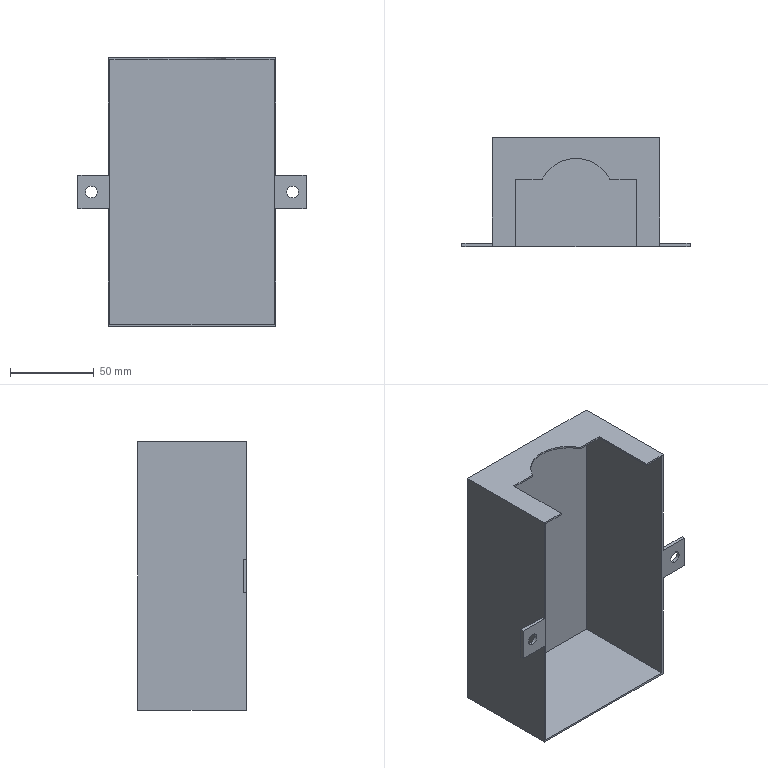Component | SolidWorks | OT-0100-029(CylinderGuard)-1 | 1 solid | 28 faces | box 136 x 65 x 160 mm | volume 47070 mm3 | plane 23 | cylinder 5 | commonest cylinder face diameters 7 x4 45 x1
build123d program:
from build123d import *

# Parameters (mm, degrees)
SKETCH1_W           = 100
SKETCH1_H           = 160
BOSS_EXTRUDE1_DEPTH = 65
SHELL1_T            = -1
SKETCH2_W           = 18
SKETCH2_H           = 20
SKETCH2_R           = 3.5
BOSS_EXTRUDE2_DEPTH = 2
CUT_EXTRUDE1_REACH  = 187.604
CUT_EXTRUDE2_START  = -1
SKETCH4_W           = 72
SKETCH4_H           = 40
CUT_EXTRUDE2_DEPTH  = 1


with BuildPart() as part:
    # Sketch1 → Boss-Extrude1 (new body)
    with BuildSketch(Plane(origin=(0, 0, 0), x_dir=(1, 0, 0), z_dir=(0, 1, 0))):
        Rectangle(SKETCH1_W, SKETCH1_H)
    extrude(amount=-BOSS_EXTRUDE1_DEPTH)

    # Shell1
    shell1_openings = [part.faces().sort_by_distance(p)[0] for p in [
        (0, -65, 0),
    ]]
    offset(amount=SHELL1_T, openings=shell1_openings, kind=Kind.INTERSECTION)

    # Sketch2 → Boss-Extrude2 (add)
    # profile 1 of 2: a face of its own
    with BuildSketch(Plane.XZ.offset(65)):
        with Locations((59, 0)):
            Rectangle(SKETCH2_W, SKETCH2_H)
        with Locations(Location((60, 0, 0), (0, 0, 270))):
            Circle(SKETCH2_R, mode=Mode.SUBTRACT)
    # profile 2 of 2: a face of its own
    with BuildSketch(Plane.XZ.offset(65)):
        with Locations((-59, 0)):
            Rectangle(SKETCH2_W, SKETCH2_H)
        with Locations(Location((-60, 0, 0), (0, 0, 90))):
            Circle(SKETCH2_R, mode=Mode.SUBTRACT)
    extrude(amount=-BOSS_EXTRUDE2_DEPTH)

    # Sketch3 → Cut-Extrude1 (cut, up to next)
    with BuildSketch(Plane.XY.offset(80), mode=Mode.PRIVATE) as cut_extrude1_sk1:
        with BuildLine():
            Line((22.5, -35), (22.5, -74.503))
            ThreePointArc((22.5, -74.503), (0, -97.003), (-22.5, -74.503))
            Line((-22.5, -74.503), (-22.5, -35))
            ThreePointArc((-22.5, -35), (0, -12.5), (22.5, -35))
        make_face()
    cut_extrude1_tool1 = extrude(cut_extrude1_sk1.sketch, amount=-CUT_EXTRUDE1_REACH, mode=Mode.PRIVATE) & part.part
    add(cut_extrude1_tool1.solids().sort_by_distance((0, -54.751, 80))[0], mode=Mode.SUBTRACT)

    # Sketch4 → Cut-Extrude2 (cut)
    with BuildSketch(Plane.XY.offset(80).offset(CUT_EXTRUDE2_START)):
        with Locations((0, -45)):
            Rectangle(SKETCH4_W, SKETCH4_H)
    extrude(amount=CUT_EXTRUDE2_DEPTH, mode=Mode.SUBTRACT)


solid = part.part

# Placed as in the assembly
solid = solid.moved(Location((200, 145, 10), (0, 0, 0)))
STEP:
#1=COLOUR_RGB('',0.7922,0.8196,0.9333);
#2=FILL_AREA_STYLE_COLOUR('',#1);
#3=FILL_AREA_STYLE('',(#2));
#4=SURFACE_STYLE_FILL_AREA(#3);
#5=SURFACE_SIDE_STYLE('',(#4));
#6=SURFACE_STYLE_USAGE(.BOTH.,#5);
#7=PRESENTATION_STYLE_ASSIGNMENT((#6));
#8=CARTESIAN_POINT('',(5.512,3.228,0.5315));
#9=VERTEX_POINT('',#8);
#10=CARTESIAN_POINT('',(5.512,3.228,0.2559));
#11=VERTEX_POINT('',#10);
#12=CARTESIAN_POINT('',(5.512,3.228,0.3937));
#13=DIRECTION('',(0.,-1.,0.));
#14=DIRECTION('',(0.,0.,1.));
#15=AXIS2_PLACEMENT_3D('',#12,#13,#14);
#16=CIRCLE('',#15,0.1378);
#17=EDGE_CURVE('',#9,#11,#16,.T.);
#18=ORIENTED_EDGE('',*,*,#17,.F.);
#19=CARTESIAN_POINT('',(5.512,3.15,0.5315));
#20=VERTEX_POINT('',#19);
#21=CARTESIAN_POINT('',(5.512,3.228,0.5315));
#22=DIRECTION('',(0.,-1.,0.));
#23=VECTOR('',#22,39.37);
#24=LINE('',#21,#23);
#25=EDGE_CURVE('',#9,#20,#24,.T.);
#26=ORIENTED_EDGE('',*,*,#25,.T.);
#27=CARTESIAN_POINT('',(5.512,3.15,0.2559));
#28=VERTEX_POINT('',#27);
#29=CARTESIAN_POINT('',(5.512,3.15,0.3937));
#30=DIRECTION('',(0.,-1.,0.));
#31=DIRECTION('',(0.,0.,1.));
#32=AXIS2_PLACEMENT_3D('',#29,#30,#31);
#33=CIRCLE('',#32,0.1378);
#34=EDGE_CURVE('',#20,#28,#33,.T.);
#35=ORIENTED_EDGE('',*,*,#34,.T.);
#36=CARTESIAN_POINT('',(5.512,3.228,0.2559));
#37=DIRECTION('',(0.,-1.,0.));
#38=VECTOR('',#37,39.37);
#39=LINE('',#36,#38);
#40=EDGE_CURVE('',#11,#28,#39,.T.);
#41=ORIENTED_EDGE('',*,*,#40,.F.);
#42=EDGE_LOOP('',(#18,#26,#35,#41));
#43=FACE_OUTER_BOUND('',#42,.T.);
#44=CARTESIAN_POINT('',(5.512,3.228,0.3937));
#45=DIRECTION('',(0.,-1.,0.));
#46=DIRECTION('',(0.,0.,-1.));
#47=AXIS2_PLACEMENT_3D('',#44,#45,#46);
#48=CYLINDRICAL_SURFACE('',#47,0.1378);
#49=ADVANCED_FACE('',(#43),#48,.F.);
#50=CARTESIAN_POINT('',(10.236,3.228,0.5315));
#51=VERTEX_POINT('',#50);
#52=CARTESIAN_POINT('',(10.236,3.228,0.2559));
#53=VERTEX_POINT('',#52);
#54=CARTESIAN_POINT('',(10.236,3.228,0.3937));
#55=DIRECTION('',(0.,-1.,0.));
#56=DIRECTION('',(0.,0.,-1.));
#57=AXIS2_PLACEMENT_3D('',#54,#55,#56);
#58=CIRCLE('',#57,0.1378);
#59=EDGE_CURVE('',#51,#53,#58,.T.);
#60=ORIENTED_EDGE('',*,*,#59,.F.);
#61=CARTESIAN_POINT('',(10.236,3.15,0.5315));
#62=VERTEX_POINT('',#61);
#63=CARTESIAN_POINT('',(10.236,3.228,0.5315));
#64=DIRECTION('',(0.,-1.,0.));
#65=VECTOR('',#64,39.37);
#66=LINE('',#63,#65);
#67=EDGE_CURVE('',#51,#62,#66,.T.);
#68=ORIENTED_EDGE('',*,*,#67,.T.);
#69=CARTESIAN_POINT('',(10.236,3.15,0.2559));
#70=VERTEX_POINT('',#69);
#71=CARTESIAN_POINT('',(10.236,3.15,0.3937));
#72=DIRECTION('',(0.,-1.,0.));
#73=DIRECTION('',(0.,0.,-1.));
#74=AXIS2_PLACEMENT_3D('',#71,#72,#73);
#75=CIRCLE('',#74,0.1378);
#76=EDGE_CURVE('',#62,#70,#75,.T.);
#77=ORIENTED_EDGE('',*,*,#76,.T.);
#78=CARTESIAN_POINT('',(10.236,3.228,0.2559));
#79=DIRECTION('',(0.,-1.,0.));
#80=VECTOR('',#79,39.37);
#81=LINE('',#78,#80);
#82=EDGE_CURVE('',#53,#70,#81,.T.);
#83=ORIENTED_EDGE('',*,*,#82,.F.);
#84=EDGE_LOOP('',(#60,#68,#77,#83));
#85=FACE_OUTER_BOUND('',#84,.T.);
#86=CARTESIAN_POINT('',(10.236,3.228,0.3937));
#87=DIRECTION('',(0.,-1.,0.));
#88=DIRECTION('',(0.,0.,-1.));
#89=AXIS2_PLACEMENT_3D('',#86,#87,#88);
#90=CYLINDRICAL_SURFACE('',#89,0.1378);
#91=ADVANCED_FACE('',(#85),#90,.F.);
#92=CARTESIAN_POINT('',(9.291,3.15,3.504));
#93=VERTEX_POINT('',#92);
#94=CARTESIAN_POINT('',(9.291,3.15,3.543));
#95=VERTEX_POINT('',#94);
#96=CARTESIAN_POINT('',(9.291,3.15,-2.756));
#97=DIRECTION('',(0.,0.,1.));
#98=VECTOR('',#97,39.37);
#99=LINE('',#96,#98);
#100=EDGE_CURVE('',#93,#95,#99,.T.);
#101=ORIENTED_EDGE('',*,*,#100,.F.);
#102=CARTESIAN_POINT('',(9.803,3.15,3.504));
#103=VERTEX_POINT('',#102);
#104=CARTESIAN_POINT('',(5.906,3.15,3.504));
#105=DIRECTION('',(1.,0.,0.));
#106=VECTOR('',#105,39.37);
#107=LINE('',#104,#106);
#108=EDGE_CURVE('',#93,#103,#107,.T.);
#109=ORIENTED_EDGE('',*,*,#108,.T.);
#110=CARTESIAN_POINT('',(9.803,3.15,-2.717));
#111=VERTEX_POINT('',#110);
#112=CARTESIAN_POINT('',(9.803,3.15,3.543));
#113=DIRECTION('',(0.,0.,-1.));
#114=VECTOR('',#113,39.37);
#115=LINE('',#112,#114);
#116=EDGE_CURVE('',#103,#111,#115,.T.);
#117=ORIENTED_EDGE('',*,*,#116,.T.);
#118=CARTESIAN_POINT('',(5.945,3.15,-2.717));
#119=VERTEX_POINT('',#118);
#120=CARTESIAN_POINT('',(5.906,3.15,-2.717));
#121=DIRECTION('',(-1.,0.,0.));
#122=VECTOR('',#121,39.37);
#123=LINE('',#120,#122);
#124=EDGE_CURVE('',#111,#119,#123,.T.);
#125=ORIENTED_EDGE('',*,*,#124,.T.);
#126=CARTESIAN_POINT('',(5.945,3.15,3.504));
#127=VERTEX_POINT('',#126);
#128=CARTESIAN_POINT('',(5.945,3.15,3.543));
#129=DIRECTION('',(0.,0.,1.));
#130=VECTOR('',#129,39.37);
#131=LINE('',#128,#130);
#132=EDGE_CURVE('',#119,#127,#131,.T.);
#133=ORIENTED_EDGE('',*,*,#132,.T.);
#134=CARTESIAN_POINT('',(6.457,3.15,3.504));
#135=VERTEX_POINT('',#134);
#136=CARTESIAN_POINT('',(5.906,3.15,3.504));
#137=DIRECTION('',(1.,0.,0.));
#138=VECTOR('',#137,39.37);
#139=LINE('',#136,#138);
#140=EDGE_CURVE('',#127,#135,#139,.T.);
#141=ORIENTED_EDGE('',*,*,#140,.T.);
#142=CARTESIAN_POINT('',(6.457,3.15,3.543));
#143=VERTEX_POINT('',#142);
#144=CARTESIAN_POINT('',(6.457,3.15,-2.756));
#145=DIRECTION('',(0.,0.,1.));
#146=VECTOR('',#145,39.37);
#147=LINE('',#144,#146);
#148=EDGE_CURVE('',#135,#143,#147,.T.);
#149=ORIENTED_EDGE('',*,*,#148,.T.);
#150=CARTESIAN_POINT('',(5.906,3.15,3.543));
#151=VERTEX_POINT('',#150);
#152=CARTESIAN_POINT('',(5.906,3.15,3.543));
#153=DIRECTION('',(1.,0.,0.));
#154=VECTOR('',#153,39.37);
#155=LINE('',#152,#154);
#156=EDGE_CURVE('',#151,#143,#155,.T.);
#157=ORIENTED_EDGE('',*,*,#156,.F.);
#158=CARTESIAN_POINT('',(5.906,3.15,0.7874));
#159=VERTEX_POINT('',#158);
#160=CARTESIAN_POINT('',(5.906,3.15,3.543));
#161=DIRECTION('',(0.,0.,1.));
#162=VECTOR('',#161,39.37);
#163=LINE('',#160,#162);
#164=EDGE_CURVE('',#159,#151,#163,.T.);
#165=ORIENTED_EDGE('',*,*,#164,.F.);
#166=CARTESIAN_POINT('',(5.197,3.15,0.7874));
#167=VERTEX_POINT('',#166);
#168=CARTESIAN_POINT('',(5.906,3.15,0.7874));
#169=DIRECTION('',(-1.,0.,-0.));
#170=VECTOR('',#169,39.37);
#171=LINE('',#168,#170);
#172=EDGE_CURVE('',#159,#167,#171,.T.);
#173=ORIENTED_EDGE('',*,*,#172,.T.);
#174=CARTESIAN_POINT('',(5.197,3.15,-0.));
#175=VERTEX_POINT('',#174);
#176=CARTESIAN_POINT('',(5.197,3.15,0.7874));
#177=DIRECTION('',(0.,0.,-1.));
#178=VECTOR('',#177,39.37);
#179=LINE('',#176,#178);
#180=EDGE_CURVE('',#167,#175,#179,.T.);
#181=ORIENTED_EDGE('',*,*,#180,.T.);
#182=CARTESIAN_POINT('',(5.906,3.15,-0.));
#183=VERTEX_POINT('',#182);
#184=CARTESIAN_POINT('',(5.906,3.15,-0.));
#185=DIRECTION('',(1.,0.,0.));
#186=VECTOR('',#185,39.37);
#187=LINE('',#184,#186);
#188=EDGE_CURVE('',#175,#183,#187,.T.);
#189=ORIENTED_EDGE('',*,*,#188,.T.);
#190=CARTESIAN_POINT('',(5.906,3.15,-2.756));
#191=VERTEX_POINT('',#190);
#192=CARTESIAN_POINT('',(5.906,3.15,3.543));
#193=DIRECTION('',(0.,0.,1.));
#194=VECTOR('',#193,39.37);
#195=LINE('',#192,#194);
#196=EDGE_CURVE('',#191,#183,#195,.T.);
#197=ORIENTED_EDGE('',*,*,#196,.F.);
#198=CARTESIAN_POINT('',(9.843,3.15,-2.756));
#199=VERTEX_POINT('',#198);
#200=CARTESIAN_POINT('',(5.906,3.15,-2.756));
#201=DIRECTION('',(-1.,0.,0.));
#202=VECTOR('',#201,39.37);
#203=LINE('',#200,#202);
#204=EDGE_CURVE('',#199,#191,#203,.T.);
#205=ORIENTED_EDGE('',*,*,#204,.F.);
#206=CARTESIAN_POINT('',(9.843,3.15,-0.));
#207=VERTEX_POINT('',#206);
#208=CARTESIAN_POINT('',(9.843,3.15,3.543));
#209=DIRECTION('',(0.,0.,-1.));
#210=VECTOR('',#209,39.37);
#211=LINE('',#208,#210);
#212=EDGE_CURVE('',#207,#199,#211,.T.);
#213=ORIENTED_EDGE('',*,*,#212,.F.);
#214=CARTESIAN_POINT('',(10.551,3.15,-0.));
#215=VERTEX_POINT('',#214);
#216=CARTESIAN_POINT('',(9.843,3.15,-0.));
#217=DIRECTION('',(1.,0.,0.));
#218=VECTOR('',#217,39.37);
#219=LINE('',#216,#218);
#220=EDGE_CURVE('',#207,#215,#219,.T.);
#221=ORIENTED_EDGE('',*,*,#220,.T.);
#222=CARTESIAN_POINT('',(10.551,3.15,0.7874));
#223=VERTEX_POINT('',#222);
#224=CARTESIAN_POINT('',(10.551,3.15,0.7874));
#225=DIRECTION('',(0.,0.,1.));
#226=VECTOR('',#225,39.37);
#227=LINE('',#224,#226);
#228=EDGE_CURVE('',#215,#223,#227,.T.);
#229=ORIENTED_EDGE('',*,*,#228,.T.);
#230=CARTESIAN_POINT('',(9.843,3.15,0.7874));
#231=VERTEX_POINT('',#230);
#232=CARTESIAN_POINT('',(9.843,3.15,0.7874));
#233=DIRECTION('',(-1.,0.,0.));
#234=VECTOR('',#233,39.37);
#235=LINE('',#232,#234);
#236=EDGE_CURVE('',#223,#231,#235,.T.);
#237=ORIENTED_EDGE('',*,*,#236,.T.);
#238=CARTESIAN_POINT('',(9.843,3.15,3.543));
#239=VERTEX_POINT('',#238);
#240=CARTESIAN_POINT('',(9.843,3.15,3.543));
#241=DIRECTION('',(0.,0.,-1.));
#242=VECTOR('',#241,39.37);
#243=LINE('',#240,#242);
#244=EDGE_CURVE('',#239,#231,#243,.T.);
#245=ORIENTED_EDGE('',*,*,#244,.F.);
#246=CARTESIAN_POINT('',(5.906,3.15,3.543));
#247=DIRECTION('',(1.,0.,0.));
#248=VECTOR('',#247,39.37);
#249=LINE('',#246,#248);
#250=EDGE_CURVE('',#95,#239,#249,.T.);
#251=ORIENTED_EDGE('',*,*,#250,.F.);
#252=EDGE_LOOP('',(#101,#109,#117,#125,#133,#141,#149,#157,#165,#173,#181,#189,#197,#205,#213,#221,#229,#237,#245,#251));
#253=FACE_OUTER_BOUND('',#252,.T.);
#254=CARTESIAN_POINT('',(10.236,3.15,0.3937));
#255=DIRECTION('',(0.,-1.,0.));
#256=DIRECTION('',(0.,0.,-1.));
#257=AXIS2_PLACEMENT_3D('',#254,#255,#256);
#258=CIRCLE('',#257,0.1378);
#259=EDGE_CURVE('',#70,#62,#258,.T.);
#260=ORIENTED_EDGE('',*,*,#259,.F.);
#261=ORIENTED_EDGE('',*,*,#76,.F.);
#262=EDGE_LOOP('',(#260,#261));
#263=FACE_BOUND('',#262,.T.);
#264=CARTESIAN_POINT('',(5.512,3.15,0.3937));
#265=DIRECTION('',(0.,-1.,0.));
#266=DIRECTION('',(0.,0.,1.));
#267=AXIS2_PLACEMENT_3D('',#264,#265,#266);
#268=CIRCLE('',#267,0.1378);
#269=EDGE_CURVE('',#28,#20,#268,.T.);
#270=ORIENTED_EDGE('',*,*,#269,.F.);
#271=ORIENTED_EDGE('',*,*,#34,.F.);
#272=EDGE_LOOP('',(#270,#271));
#273=FACE_BOUND('',#272,.T.);
#274=CARTESIAN_POINT('',(7.874,3.15,0.3937));
#275=DIRECTION('',(0.,-1.,0.));
#276=DIRECTION('',(0.,0.,-1.));
#277=AXIS2_PLACEMENT_3D('',#274,#275,#276);
#278=PLANE('',#277);
#279=ADVANCED_FACE('',(#253,#263,#273),#278,.T.);
#280=CARTESIAN_POINT('',(9.843,3.228,0.7874));
#281=VERTEX_POINT('',#280);
#282=CARTESIAN_POINT('',(9.843,3.228,0.7874));
#283=DIRECTION('',(0.,-1.,0.));
#284=VECTOR('',#283,39.37);
#285=LINE('',#282,#284);
#286=EDGE_CURVE('',#281,#231,#285,.T.);
#287=ORIENTED_EDGE('',*,*,#286,.F.);
#288=CARTESIAN_POINT('',(9.843,3.228,-0.));
#289=VERTEX_POINT('',#288);
#290=CARTESIAN_POINT('',(9.843,3.228,0.7874));
#291=DIRECTION('',(0.,0.,-1.));
#292=VECTOR('',#291,39.37);
#293=LINE('',#290,#292);
#294=EDGE_CURVE('',#281,#289,#293,.T.);
#295=ORIENTED_EDGE('',*,*,#294,.T.);
#296=CARTESIAN_POINT('',(9.843,3.228,-0.));
#297=DIRECTION('',(0.,-1.,0.));
#298=VECTOR('',#297,39.37);
#299=LINE('',#296,#298);
#300=EDGE_CURVE('',#289,#207,#299,.T.);
#301=ORIENTED_EDGE('',*,*,#300,.T.);
#302=ORIENTED_EDGE('',*,*,#212,.T.);
#303=CARTESIAN_POINT('',(9.843,5.709,-2.756));
#304=VERTEX_POINT('',#303);
#305=CARTESIAN_POINT('',(9.843,3.15,-2.756));
#306=DIRECTION('',(0.,1.,0.));
#307=VECTOR('',#306,39.37);
#308=LINE('',#305,#307);
#309=EDGE_CURVE('',#199,#304,#308,.T.);
#310=ORIENTED_EDGE('',*,*,#309,.T.);
#311=CARTESIAN_POINT('',(9.843,5.709,3.543));
#312=VERTEX_POINT('',#311);
#313=CARTESIAN_POINT('',(9.843,5.709,3.543));
#314=DIRECTION('',(0.,0.,-1.));
#315=VECTOR('',#314,39.37);
#316=LINE('',#313,#315);
#317=EDGE_CURVE('',#312,#304,#316,.T.);
#318=ORIENTED_EDGE('',*,*,#317,.F.);
#319=CARTESIAN_POINT('',(9.843,3.15,3.543));
#320=DIRECTION('',(0.,1.,0.));
#321=VECTOR('',#320,39.37);
#322=LINE('',#319,#321);
#323=EDGE_CURVE('',#239,#312,#322,.T.);
#324=ORIENTED_EDGE('',*,*,#323,.F.);
#325=ORIENTED_EDGE('',*,*,#244,.T.);
#326=EDGE_LOOP('',(#287,#295,#301,#302,#310,#318,#324,#325));
#327=FACE_OUTER_BOUND('',#326,.T.);
#328=CARTESIAN_POINT('',(9.843,3.15,3.543));
#329=DIRECTION('',(1.,0.,0.));
#330=DIRECTION('',(0.,0.,-1.));
#331=AXIS2_PLACEMENT_3D('',#328,#329,#330);
#332=PLANE('',#331);
#333=ADVANCED_FACE('',(#327),#332,.T.);
#334=CARTESIAN_POINT('',(9.291,4.724,3.543));
#335=VERTEX_POINT('',#334);
#336=CARTESIAN_POINT('',(8.668,4.724,3.543));
#337=VERTEX_POINT('',#336);
#338=CARTESIAN_POINT('',(6.457,4.724,3.543));
#339=DIRECTION('',(-1.,0.,0.));
#340=VECTOR('',#339,39.37);
#341=LINE('',#338,#340);
#342=EDGE_CURVE('',#335,#337,#341,.T.);
#343=ORIENTED_EDGE('',*,*,#342,.F.);
#344=CARTESIAN_POINT('',(9.291,3.15,3.543));
#345=DIRECTION('',(0.,1.,0.));
#346=VECTOR('',#345,39.37);
#347=LINE('',#344,#346);
#348=EDGE_CURVE('',#95,#335,#347,.T.);
#349=ORIENTED_EDGE('',*,*,#348,.F.);
#350=ORIENTED_EDGE('',*,*,#250,.T.);
#351=ORIENTED_EDGE('',*,*,#323,.T.);
#352=CARTESIAN_POINT('',(5.906,5.709,3.543));
#353=VERTEX_POINT('',#352);
#354=CARTESIAN_POINT('',(5.906,5.709,3.543));
#355=DIRECTION('',(1.,0.,0.));
#356=VECTOR('',#355,39.37);
#357=LINE('',#354,#356);
#358=EDGE_CURVE('',#353,#312,#357,.T.);
#359=ORIENTED_EDGE('',*,*,#358,.F.);
#360=CARTESIAN_POINT('',(5.906,3.15,3.543));
#361=DIRECTION('',(0.,1.,0.));
#362=VECTOR('',#361,39.37);
#363=LINE('',#360,#362);
#364=EDGE_CURVE('',#151,#353,#363,.T.);
#365=ORIENTED_EDGE('',*,*,#364,.F.);
#366=ORIENTED_EDGE('',*,*,#156,.T.);
#367=CARTESIAN_POINT('',(6.457,4.724,3.543));
#368=VERTEX_POINT('',#367);
#369=CARTESIAN_POINT('',(6.457,3.15,3.543));
#370=DIRECTION('',(0.,-1.,0.));
#371=VECTOR('',#370,39.37);
#372=LINE('',#369,#371);
#373=EDGE_CURVE('',#368,#143,#372,.T.);
#374=ORIENTED_EDGE('',*,*,#373,.F.);
#375=CARTESIAN_POINT('',(7.08,4.724,3.543));
#376=VERTEX_POINT('',#375);
#377=CARTESIAN_POINT('',(6.457,4.724,3.543));
#378=DIRECTION('',(-1.,0.,0.));
#379=VECTOR('',#378,39.37);
#380=LINE('',#377,#379);
#381=EDGE_CURVE('',#376,#368,#380,.T.);
#382=ORIENTED_EDGE('',*,*,#381,.F.);
#383=CARTESIAN_POINT('',(7.874,4.331,3.543));
#384=DIRECTION('',(0.,0.,1.));
#385=DIRECTION('',(1.,0.,0.));
#386=AXIS2_PLACEMENT_3D('',#383,#384,#385);
#387=CIRCLE('',#386,0.8858);
#388=EDGE_CURVE('',#337,#376,#387,.T.);
#389=ORIENTED_EDGE('',*,*,#388,.F.);
#390=EDGE_LOOP('',(#343,#349,#350,#351,#359,#365,#366,#374,#382,#389));
#391=FACE_OUTER_BOUND('',#390,.T.);
#392=CARTESIAN_POINT('',(5.906,3.15,3.543));
#393=DIRECTION('',(0.,0.,1.));
#394=DIRECTION('',(1.,0.,0.));
#395=AXIS2_PLACEMENT_3D('',#392,#393,#394);
#396=PLANE('',#395);
#397=ADVANCED_FACE('',(#391),#396,.T.);
#398=CARTESIAN_POINT('',(5.906,3.228,-0.));
#399=VERTEX_POINT('',#398);
#400=CARTESIAN_POINT('',(5.906,3.228,-0.));
#401=DIRECTION('',(0.,-1.,0.));
#402=VECTOR('',#401,39.37);
#403=LINE('',#400,#402);
#404=EDGE_CURVE('',#399,#183,#403,.T.);
#405=ORIENTED_EDGE('',*,*,#404,.F.);
#406=CARTESIAN_POINT('',(5.906,3.228,0.7874));
#407=VERTEX_POINT('',#406);
#408=CARTESIAN_POINT('',(5.906,3.228,0.7874));
#409=DIRECTION('',(0.,0.,1.));
#410=VECTOR('',#409,39.37);
#411=LINE('',#408,#410);
#412=EDGE_CURVE('',#399,#407,#411,.T.);
#413=ORIENTED_EDGE('',*,*,#412,.T.);
#414=CARTESIAN_POINT('',(5.906,3.228,0.7874));
#415=DIRECTION('',(0.,-1.,0.));
#416=VECTOR('',#415,39.37);
#417=LINE('',#414,#416);
#418=EDGE_CURVE('',#407,#159,#417,.T.);
#419=ORIENTED_EDGE('',*,*,#418,.T.);
#420=ORIENTED_EDGE('',*,*,#164,.T.);
#421=ORIENTED_EDGE('',*,*,#364,.T.);
#422=CARTESIAN_POINT('',(5.906,5.709,-2.756));
#423=VERTEX_POINT('',#422);
#424=CARTESIAN_POINT('',(5.906,5.709,3.543));
#425=DIRECTION('',(0.,0.,1.));
#426=VECTOR('',#425,39.37);
#427=LINE('',#424,#426);
#428=EDGE_CURVE('',#423,#353,#427,.T.);
#429=ORIENTED_EDGE('',*,*,#428,.F.);
#430=CARTESIAN_POINT('',(5.906,3.15,-2.756));
#431=DIRECTION('',(0.,1.,0.));
#432=VECTOR('',#431,39.37);
#433=LINE('',#430,#432);
#434=EDGE_CURVE('',#191,#423,#433,.T.);
#435=ORIENTED_EDGE('',*,*,#434,.F.);
#436=ORIENTED_EDGE('',*,*,#196,.T.);
#437=EDGE_LOOP('',(#405,#413,#419,#420,#421,#429,#435,#436));
#438=FACE_OUTER_BOUND('',#437,.T.);
#439=CARTESIAN_POINT('',(5.906,3.15,3.543));
#440=DIRECTION('',(-1.,0.,0.));
#441=DIRECTION('',(0.,0.,1.));
#442=AXIS2_PLACEMENT_3D('',#439,#440,#441);
#443=PLANE('',#442);
#444=ADVANCED_FACE('',(#438),#443,.T.);
#445=CARTESIAN_POINT('',(5.906,5.709,-2.756));
#446=DIRECTION('',(-1.,0.,0.));
#447=VECTOR('',#446,39.37);
#448=LINE('',#445,#447);
#449=EDGE_CURVE('',#304,#423,#448,.T.);
#450=ORIENTED_EDGE('',*,*,#449,.F.);
#451=ORIENTED_EDGE('',*,*,#309,.F.);
#452=ORIENTED_EDGE('',*,*,#204,.T.);
#453=ORIENTED_EDGE('',*,*,#434,.T.);
#454=EDGE_LOOP('',(#450,#451,#452,#453));
#455=FACE_OUTER_BOUND('',#454,.T.);
#456=CARTESIAN_POINT('',(5.906,3.15,-2.756));
#457=DIRECTION('',(0.,0.,-1.));
#458=DIRECTION('',(-1.,0.,0.));
#459=AXIS2_PLACEMENT_3D('',#456,#457,#458);
#460=PLANE('',#459);
#461=ADVANCED_FACE('',(#455),#460,.T.);
#462=ORIENTED_EDGE('',*,*,#317,.T.);
#463=ORIENTED_EDGE('',*,*,#449,.T.);
#464=ORIENTED_EDGE('',*,*,#428,.T.);
#465=ORIENTED_EDGE('',*,*,#358,.T.);
#466=EDGE_LOOP('',(#462,#463,#464,#465));
#467=FACE_OUTER_BOUND('',#466,.T.);
#468=CARTESIAN_POINT('',(7.874,5.709,0.3937));
#469=DIRECTION('',(0.,-1.,0.));
#470=DIRECTION('',(0.,0.,-1.));
#471=AXIS2_PLACEMENT_3D('',#468,#469,#470);
#472=PLANE('',#471);
#473=ADVANCED_FACE('',(#467),#472,.F.);
#474=CARTESIAN_POINT('',(9.803,5.669,3.504));
#475=VERTEX_POINT('',#474);
#476=CARTESIAN_POINT('',(9.803,5.669,-2.717));
#477=VERTEX_POINT('',#476);
#478=CARTESIAN_POINT('',(9.803,5.669,3.543));
#479=DIRECTION('',(0.,0.,-1.));
#480=VECTOR('',#479,39.37);
#481=LINE('',#478,#480);
#482=EDGE_CURVE('',#475,#477,#481,.T.);
#483=ORIENTED_EDGE('',*,*,#482,.T.);
#484=CARTESIAN_POINT('',(9.803,3.15,-2.717));
#485=DIRECTION('',(0.,1.,0.));
#486=VECTOR('',#485,39.37);
#487=LINE('',#484,#486);
#488=EDGE_CURVE('',#111,#477,#487,.T.);
#489=ORIENTED_EDGE('',*,*,#488,.F.);
#490=ORIENTED_EDGE('',*,*,#116,.F.);
#491=CARTESIAN_POINT('',(9.803,3.15,3.504));
#492=DIRECTION('',(0.,1.,0.));
#493=VECTOR('',#492,39.37);
#494=LINE('',#491,#493);
#495=EDGE_CURVE('',#103,#475,#494,.T.);
#496=ORIENTED_EDGE('',*,*,#495,.T.);
#497=EDGE_LOOP('',(#483,#489,#490,#496));
#498=FACE_OUTER_BOUND('',#497,.T.);
#499=CARTESIAN_POINT('',(9.803,3.15,3.543));
#500=DIRECTION('',(1.,0.,0.));
#501=DIRECTION('',(0.,0.,-1.));
#502=AXIS2_PLACEMENT_3D('',#499,#500,#501);
#503=PLANE('',#502);
#504=ADVANCED_FACE('',(#498),#503,.F.);
#505=CARTESIAN_POINT('',(9.291,4.724,3.504));
#506=VERTEX_POINT('',#505);
#507=CARTESIAN_POINT('',(9.291,3.15,3.504));
#508=DIRECTION('',(0.,-1.,0.));
#509=VECTOR('',#508,39.37);
#510=LINE('',#507,#509);
#511=EDGE_CURVE('',#506,#93,#510,.T.);
#512=ORIENTED_EDGE('',*,*,#511,.F.);
#513=CARTESIAN_POINT('',(8.668,4.724,3.504));
#514=VERTEX_POINT('',#513);
#515=CARTESIAN_POINT('',(6.457,4.724,3.504));
#516=DIRECTION('',(1.,0.,0.));
#517=VECTOR('',#516,39.37);
#518=LINE('',#515,#517);
#519=EDGE_CURVE('',#514,#506,#518,.T.);
#520=ORIENTED_EDGE('',*,*,#519,.F.);
#521=CARTESIAN_POINT('',(7.08,4.724,3.504));
#522=VERTEX_POINT('',#521);
#523=CARTESIAN_POINT('',(7.874,4.331,3.504));
#524=DIRECTION('',(0.,0.,-1.));
#525=DIRECTION('',(1.,0.,0.));
#526=AXIS2_PLACEMENT_3D('',#523,#524,#525);
#527=CIRCLE('',#526,0.8858);
#528=EDGE_CURVE('',#522,#514,#527,.T.);
#529=ORIENTED_EDGE('',*,*,#528,.F.);
#530=CARTESIAN_POINT('',(6.457,4.724,3.504));
#531=VERTEX_POINT('',#530);
#532=CARTESIAN_POINT('',(6.457,4.724,3.504));
#533=DIRECTION('',(1.,0.,0.));
#534=VECTOR('',#533,39.37);
#535=LINE('',#532,#534);
#536=EDGE_CURVE('',#531,#522,#535,.T.);
#537=ORIENTED_EDGE('',*,*,#536,.F.);
#538=CARTESIAN_POINT('',(6.457,3.15,3.504));
#539=DIRECTION('',(0.,1.,0.));
#540=VECTOR('',#539,39.37);
#541=LINE('',#538,#540);
#542=EDGE_CURVE('',#135,#531,#541,.T.);
#543=ORIENTED_EDGE('',*,*,#542,.F.);
#544=ORIENTED_EDGE('',*,*,#140,.F.);
#545=CARTESIAN_POINT('',(5.945,5.669,3.504));
#546=VERTEX_POINT('',#545);
#547=CARTESIAN_POINT('',(5.945,3.15,3.504));
#548=DIRECTION('',(0.,1.,0.));
#549=VECTOR('',#548,39.37);
#550=LINE('',#547,#549);
#551=EDGE_CURVE('',#127,#546,#550,.T.);
#552=ORIENTED_EDGE('',*,*,#551,.T.);
#553=CARTESIAN_POINT('',(5.906,5.669,3.504));
#554=DIRECTION('',(1.,0.,0.));
#555=VECTOR('',#554,39.37);
#556=LINE('',#553,#555);
#557=EDGE_CURVE('',#546,#475,#556,.T.);
#558=ORIENTED_EDGE('',*,*,#557,.T.);
#559=ORIENTED_EDGE('',*,*,#495,.F.);
#560=ORIENTED_EDGE('',*,*,#108,.F.);
#561=EDGE_LOOP('',(#512,#520,#529,#537,#543,#544,#552,#558,#559,#560));
#562=FACE_OUTER_BOUND('',#561,.T.);
#563=CARTESIAN_POINT('',(5.906,3.15,3.504));
#564=DIRECTION('',(0.,0.,1.));
#565=DIRECTION('',(1.,0.,0.));
#566=AXIS2_PLACEMENT_3D('',#563,#564,#565);
#567=PLANE('',#566);
#568=ADVANCED_FACE('',(#562),#567,.F.);
#569=CARTESIAN_POINT('',(5.945,5.669,-2.717));
#570=VERTEX_POINT('',#569);
#571=CARTESIAN_POINT('',(5.945,5.669,3.543));
#572=DIRECTION('',(0.,0.,1.));
#573=VECTOR('',#572,39.37);
#574=LINE('',#571,#573);
#575=EDGE_CURVE('',#570,#546,#574,.T.);
#576=ORIENTED_EDGE('',*,*,#575,.T.);
#577=ORIENTED_EDGE('',*,*,#551,.F.);
#578=ORIENTED_EDGE('',*,*,#132,.F.);
#579=CARTESIAN_POINT('',(5.945,3.15,-2.717));
#580=DIRECTION('',(0.,1.,0.));
#581=VECTOR('',#580,39.37);
#582=LINE('',#579,#581);
#583=EDGE_CURVE('',#119,#570,#582,.T.);
#584=ORIENTED_EDGE('',*,*,#583,.T.);
#585=EDGE_LOOP('',(#576,#577,#578,#584));
#586=FACE_OUTER_BOUND('',#585,.T.);
#587=CARTESIAN_POINT('',(5.945,3.15,3.543));
#588=DIRECTION('',(-1.,0.,0.));
#589=DIRECTION('',(0.,0.,1.));
#590=AXIS2_PLACEMENT_3D('',#587,#588,#589);
#591=PLANE('',#590);
#592=ADVANCED_FACE('',(#586),#591,.F.);
#593=CARTESIAN_POINT('',(5.906,5.669,-2.717));
#594=DIRECTION('',(-1.,0.,0.));
#595=VECTOR('',#594,39.37);
#596=LINE('',#593,#595);
#597=EDGE_CURVE('',#477,#570,#596,.T.);
#598=ORIENTED_EDGE('',*,*,#597,.T.);
#599=ORIENTED_EDGE('',*,*,#583,.F.);
#600=ORIENTED_EDGE('',*,*,#124,.F.);
#601=ORIENTED_EDGE('',*,*,#488,.T.);
#602=EDGE_LOOP('',(#598,#599,#600,#601));
#603=FACE_OUTER_BOUND('',#602,.T.);
#604=CARTESIAN_POINT('',(5.906,3.15,-2.717));
#605=DIRECTION('',(0.,0.,-1.));
#606=DIRECTION('',(-1.,0.,0.));
#607=AXIS2_PLACEMENT_3D('',#604,#605,#606);
#608=PLANE('',#607);
#609=ADVANCED_FACE('',(#603),#608,.F.);
#610=ORIENTED_EDGE('',*,*,#482,.F.);
#611=ORIENTED_EDGE('',*,*,#557,.F.);
#612=ORIENTED_EDGE('',*,*,#575,.F.);
#613=ORIENTED_EDGE('',*,*,#597,.F.);
#614=EDGE_LOOP('',(#610,#611,#612,#613));
#615=FACE_OUTER_BOUND('',#614,.T.);
#616=CARTESIAN_POINT('',(7.874,5.669,0.3937));
#617=DIRECTION('',(0.,-1.,0.));
#618=DIRECTION('',(0.,0.,-1.));
#619=AXIS2_PLACEMENT_3D('',#616,#617,#618);
#620=PLANE('',#619);
#621=ADVANCED_FACE('',(#615),#620,.T.);
#622=ORIENTED_EDGE('',*,*,#236,.F.);
#623=CARTESIAN_POINT('',(10.551,3.228,0.7874));
#624=VERTEX_POINT('',#623);
#625=CARTESIAN_POINT('',(10.551,3.228,0.7874));
#626=DIRECTION('',(0.,-1.,0.));
#627=VECTOR('',#626,39.37);
#628=LINE('',#625,#627);
#629=EDGE_CURVE('',#624,#223,#628,.T.);
#630=ORIENTED_EDGE('',*,*,#629,.F.);
#631=CARTESIAN_POINT('',(9.843,3.228,0.7874));
#632=DIRECTION('',(-1.,0.,0.));
#633=VECTOR('',#632,39.37);
#634=LINE('',#631,#633);
#635=EDGE_CURVE('',#624,#281,#634,.T.);
#636=ORIENTED_EDGE('',*,*,#635,.T.);
#637=ORIENTED_EDGE('',*,*,#286,.T.);
#638=EDGE_LOOP('',(#622,#630,#636,#637));
#639=FACE_OUTER_BOUND('',#638,.T.);
#640=CARTESIAN_POINT('',(9.843,3.228,0.7874));
#641=DIRECTION('',(0.,0.,1.));
#642=DIRECTION('',(1.,0.,-0.));
#643=AXIS2_PLACEMENT_3D('',#640,#641,#642);
#644=PLANE('',#643);
#645=ADVANCED_FACE('',(#639),#644,.T.);
#646=ORIENTED_EDGE('',*,*,#228,.F.);
#647=CARTESIAN_POINT('',(10.551,3.228,-0.));
#648=VERTEX_POINT('',#647);
#649=CARTESIAN_POINT('',(10.551,3.228,-0.));
#650=DIRECTION('',(0.,-1.,0.));
#651=VECTOR('',#650,39.37);
#652=LINE('',#649,#651);
#653=EDGE_CURVE('',#648,#215,#652,.T.);
#654=ORIENTED_EDGE('',*,*,#653,.F.);
#655=CARTESIAN_POINT('',(10.551,3.228,0.7874));
#656=DIRECTION('',(0.,0.,1.));
#657=VECTOR('',#656,39.37);
#658=LINE('',#655,#657);
#659=EDGE_CURVE('',#648,#624,#658,.T.);
#660=ORIENTED_EDGE('',*,*,#659,.T.);
#661=ORIENTED_EDGE('',*,*,#629,.T.);
#662=EDGE_LOOP('',(#646,#654,#660,#661));
#663=FACE_OUTER_BOUND('',#662,.T.);
#664=CARTESIAN_POINT('',(10.551,3.228,0.7874));
#665=DIRECTION('',(1.,0.,0.));
#666=DIRECTION('',(0.,0.,-1.));
#667=AXIS2_PLACEMENT_3D('',#664,#665,#666);
#668=PLANE('',#667);
#669=ADVANCED_FACE('',(#663),#668,.T.);
#670=ORIENTED_EDGE('',*,*,#220,.F.);
#671=ORIENTED_EDGE('',*,*,#300,.F.);
#672=CARTESIAN_POINT('',(9.843,3.228,-0.));
#673=DIRECTION('',(1.,0.,0.));
#674=VECTOR('',#673,39.37);
#675=LINE('',#672,#674);
#676=EDGE_CURVE('',#289,#648,#675,.T.);
#677=ORIENTED_EDGE('',*,*,#676,.T.);
#678=ORIENTED_EDGE('',*,*,#653,.T.);
#679=EDGE_LOOP('',(#670,#671,#677,#678));
#680=FACE_OUTER_BOUND('',#679,.T.);
#681=CARTESIAN_POINT('',(9.843,3.228,-0.));
#682=DIRECTION('',(0.,0.,-1.));
#683=DIRECTION('',(-1.,0.,0.));
#684=AXIS2_PLACEMENT_3D('',#681,#682,#683);
#685=PLANE('',#684);
#686=ADVANCED_FACE('',(#680),#685,.T.);
#687=CARTESIAN_POINT('',(10.236,3.228,0.3937));
#688=DIRECTION('',(0.,-1.,0.));
#689=DIRECTION('',(0.,0.,-1.));
#690=AXIS2_PLACEMENT_3D('',#687,#688,#689);
#691=CIRCLE('',#690,0.1378);
#692=EDGE_CURVE('',#53,#51,#691,.T.);
#693=ORIENTED_EDGE('',*,*,#692,.T.);
#694=ORIENTED_EDGE('',*,*,#59,.T.);
#695=EDGE_LOOP('',(#693,#694));
#696=FACE_BOUND('',#695,.T.);
#697=ORIENTED_EDGE('',*,*,#294,.F.);
#698=ORIENTED_EDGE('',*,*,#635,.F.);
#699=ORIENTED_EDGE('',*,*,#659,.F.);
#700=ORIENTED_EDGE('',*,*,#676,.F.);
#701=EDGE_LOOP('',(#697,#698,#699,#700));
#702=FACE_OUTER_BOUND('',#701,.T.);
#703=CARTESIAN_POINT('',(7.874,3.228,0.3937));
#704=DIRECTION('',(0.,-1.,0.));
#705=DIRECTION('',(0.,0.,-1.));
#706=AXIS2_PLACEMENT_3D('',#703,#704,#705);
#707=PLANE('',#706);
#708=ADVANCED_FACE('',(#696,#702),#707,.F.);
#709=ORIENTED_EDGE('',*,*,#67,.F.);
#710=ORIENTED_EDGE('',*,*,#692,.F.);
#711=ORIENTED_EDGE('',*,*,#82,.T.);
#712=ORIENTED_EDGE('',*,*,#259,.T.);
#713=EDGE_LOOP('',(#709,#710,#711,#712));
#714=FACE_OUTER_BOUND('',#713,.T.);
#715=CARTESIAN_POINT('',(10.236,3.228,0.3937));
#716=DIRECTION('',(0.,-1.,0.));
#717=DIRECTION('',(0.,0.,-1.));
#718=AXIS2_PLACEMENT_3D('',#715,#716,#717);
#719=CYLINDRICAL_SURFACE('',#718,0.1378);
#720=ADVANCED_FACE('',(#714),#719,.F.);
#721=ORIENTED_EDGE('',*,*,#172,.F.);
#722=ORIENTED_EDGE('',*,*,#418,.F.);
#723=CARTESIAN_POINT('',(5.197,3.228,0.7874));
#724=VERTEX_POINT('',#723);
#725=CARTESIAN_POINT('',(5.906,3.228,0.7874));
#726=DIRECTION('',(-1.,0.,-0.));
#727=VECTOR('',#726,39.37);
#728=LINE('',#725,#727);
#729=EDGE_CURVE('',#407,#724,#728,.T.);
#730=ORIENTED_EDGE('',*,*,#729,.T.);
#731=CARTESIAN_POINT('',(5.197,3.228,0.7874));
#732=DIRECTION('',(0.,-1.,0.));
#733=VECTOR('',#732,39.37);
#734=LINE('',#731,#733);
#735=EDGE_CURVE('',#724,#167,#734,.T.);
#736=ORIENTED_EDGE('',*,*,#735,.T.);
#737=EDGE_LOOP('',(#721,#722,#730,#736));
#738=FACE_OUTER_BOUND('',#737,.T.);
#739=CARTESIAN_POINT('',(5.906,3.228,0.7874));
#740=DIRECTION('',(-0.,0.,1.));
#741=DIRECTION('',(1.,0.,0.));
#742=AXIS2_PLACEMENT_3D('',#739,#740,#741);
#743=PLANE('',#742);
#744=ADVANCED_FACE('',(#738),#743,.T.);
#745=ORIENTED_EDGE('',*,*,#188,.F.);
#746=CARTESIAN_POINT('',(5.197,3.228,-0.));
#747=VERTEX_POINT('',#746);
#748=CARTESIAN_POINT('',(5.197,3.228,-0.));
#749=DIRECTION('',(0.,-1.,0.));
#750=VECTOR('',#749,39.37);
#751=LINE('',#748,#750);
#752=EDGE_CURVE('',#747,#175,#751,.T.);
#753=ORIENTED_EDGE('',*,*,#752,.F.);
#754=CARTESIAN_POINT('',(5.906,3.228,-0.));
#755=DIRECTION('',(1.,0.,0.));
#756=VECTOR('',#755,39.37);
#757=LINE('',#754,#756);
#758=EDGE_CURVE('',#747,#399,#757,.T.);
#759=ORIENTED_EDGE('',*,*,#758,.T.);
#760=ORIENTED_EDGE('',*,*,#404,.T.);
#761=EDGE_LOOP('',(#745,#753,#759,#760));
#762=FACE_OUTER_BOUND('',#761,.T.);
#763=CARTESIAN_POINT('',(5.906,3.228,-0.));
#764=DIRECTION('',(0.,0.,-1.));
#765=DIRECTION('',(-1.,0.,0.));
#766=AXIS2_PLACEMENT_3D('',#763,#764,#765);
#767=PLANE('',#766);
#768=ADVANCED_FACE('',(#762),#767,.T.);
#769=ORIENTED_EDGE('',*,*,#180,.F.);
#770=ORIENTED_EDGE('',*,*,#735,.F.);
#771=CARTESIAN_POINT('',(5.197,3.228,0.7874));
#772=DIRECTION('',(0.,0.,-1.));
#773=VECTOR('',#772,39.37);
#774=LINE('',#771,#773);
#775=EDGE_CURVE('',#724,#747,#774,.T.);
#776=ORIENTED_EDGE('',*,*,#775,.T.);
#777=ORIENTED_EDGE('',*,*,#752,.T.);
#778=EDGE_LOOP('',(#769,#770,#776,#777));
#779=FACE_OUTER_BOUND('',#778,.T.);
#780=CARTESIAN_POINT('',(5.197,3.228,0.7874));
#781=DIRECTION('',(-1.,0.,0.));
#782=DIRECTION('',(0.,0.,1.));
#783=AXIS2_PLACEMENT_3D('',#780,#781,#782);
#784=PLANE('',#783);
#785=ADVANCED_FACE('',(#779),#784,.T.);
#786=CARTESIAN_POINT('',(5.512,3.228,0.3937));
#787=DIRECTION('',(0.,-1.,0.));
#788=DIRECTION('',(0.,0.,1.));
#789=AXIS2_PLACEMENT_3D('',#786,#787,#788);
#790=CIRCLE('',#789,0.1378);
#791=EDGE_CURVE('',#11,#9,#790,.T.);
#792=ORIENTED_EDGE('',*,*,#791,.T.);
#793=ORIENTED_EDGE('',*,*,#17,.T.);
#794=EDGE_LOOP('',(#792,#793));
#795=FACE_BOUND('',#794,.T.);
#796=ORIENTED_EDGE('',*,*,#729,.F.);
#797=ORIENTED_EDGE('',*,*,#412,.F.);
#798=ORIENTED_EDGE('',*,*,#758,.F.);
#799=ORIENTED_EDGE('',*,*,#775,.F.);
#800=EDGE_LOOP('',(#796,#797,#798,#799));
#801=FACE_OUTER_BOUND('',#800,.T.);
#802=CARTESIAN_POINT('',(7.874,3.228,0.3937));
#803=DIRECTION('',(0.,-1.,0.));
#804=DIRECTION('',(0.,0.,-1.));
#805=AXIS2_PLACEMENT_3D('',#802,#803,#804);
#806=PLANE('',#805);
#807=ADVANCED_FACE('',(#795,#801),#806,.F.);
#808=ORIENTED_EDGE('',*,*,#25,.F.);
#809=ORIENTED_EDGE('',*,*,#791,.F.);
#810=ORIENTED_EDGE('',*,*,#40,.T.);
#811=ORIENTED_EDGE('',*,*,#269,.T.);
#812=EDGE_LOOP('',(#808,#809,#810,#811));
#813=FACE_OUTER_BOUND('',#812,.T.);
#814=CARTESIAN_POINT('',(5.512,3.228,0.3937));
#815=DIRECTION('',(0.,-1.,0.));
#816=DIRECTION('',(0.,0.,-1.));
#817=AXIS2_PLACEMENT_3D('',#814,#815,#816);
#818=CYLINDRICAL_SURFACE('',#817,0.1378);
#819=ADVANCED_FACE('',(#813),#818,.F.);
#820=ORIENTED_EDGE('',*,*,#528,.T.);
#821=CARTESIAN_POINT('',(8.668,4.724,-2.756));
#822=DIRECTION('',(0.,0.,-1.));
#823=VECTOR('',#822,39.37);
#824=LINE('',#821,#823);
#825=EDGE_CURVE('',#337,#514,#824,.T.);
#826=ORIENTED_EDGE('',*,*,#825,.F.);
#827=ORIENTED_EDGE('',*,*,#388,.T.);
#828=CARTESIAN_POINT('',(7.08,4.724,-2.756));
#829=DIRECTION('',(0.,0.,1.));
#830=VECTOR('',#829,39.37);
#831=LINE('',#828,#830);
#832=EDGE_CURVE('',#522,#376,#831,.T.);
#833=ORIENTED_EDGE('',*,*,#832,.F.);
#834=EDGE_LOOP('',(#820,#826,#827,#833));
#835=FACE_OUTER_BOUND('',#834,.T.);
#836=CARTESIAN_POINT('',(7.874,4.331,-2.756));
#837=DIRECTION('',(0.,0.,1.));
#838=DIRECTION('',(1.,0.,0.));
#839=AXIS2_PLACEMENT_3D('',#836,#837,#838);
#840=CYLINDRICAL_SURFACE('',#839,0.8858);
#841=ADVANCED_FACE('',(#835),#840,.F.);
#842=ORIENTED_EDGE('',*,*,#536,.T.);
#843=ORIENTED_EDGE('',*,*,#832,.T.);
#844=ORIENTED_EDGE('',*,*,#381,.T.);
#845=CARTESIAN_POINT('',(6.457,4.724,-2.756));
#846=DIRECTION('',(0.,0.,1.));
#847=VECTOR('',#846,39.37);
#848=LINE('',#845,#847);
#849=EDGE_CURVE('',#531,#368,#848,.T.);
#850=ORIENTED_EDGE('',*,*,#849,.F.);
#851=EDGE_LOOP('',(#842,#843,#844,#850));
#852=FACE_OUTER_BOUND('',#851,.T.);
#853=CARTESIAN_POINT('',(6.457,4.724,-2.756));
#854=DIRECTION('',(0.,1.,0.));
#855=DIRECTION('',(0.,0.,1.));
#856=AXIS2_PLACEMENT_3D('',#853,#854,#855);
#857=PLANE('',#856);
#858=ADVANCED_FACE('',(#852),#857,.F.);
#859=ORIENTED_EDGE('',*,*,#542,.T.);
#860=ORIENTED_EDGE('',*,*,#849,.T.);
#861=ORIENTED_EDGE('',*,*,#373,.T.);
#862=ORIENTED_EDGE('',*,*,#148,.F.);
#863=EDGE_LOOP('',(#859,#860,#861,#862));
#864=FACE_OUTER_BOUND('',#863,.T.);
#865=CARTESIAN_POINT('',(6.457,3.15,-2.756));
#866=DIRECTION('',(-1.,0.,0.));
#867=DIRECTION('',(0.,0.,1.));
#868=AXIS2_PLACEMENT_3D('',#865,#866,#867);
#869=PLANE('',#868);
#870=ADVANCED_FACE('',(#864),#869,.F.);
#871=ORIENTED_EDGE('',*,*,#519,.T.);
#872=CARTESIAN_POINT('',(9.291,4.724,-2.756));
#873=DIRECTION('',(0.,0.,1.));
#874=VECTOR('',#873,39.37);
#875=LINE('',#872,#874);
#876=EDGE_CURVE('',#506,#335,#875,.T.);
#877=ORIENTED_EDGE('',*,*,#876,.T.);
#878=ORIENTED_EDGE('',*,*,#342,.T.);
#879=ORIENTED_EDGE('',*,*,#825,.T.);
#880=EDGE_LOOP('',(#871,#877,#878,#879));
#881=FACE_OUTER_BOUND('',#880,.T.);
#882=CARTESIAN_POINT('',(6.457,4.724,-2.756));
#883=DIRECTION('',(0.,1.,0.));
#884=DIRECTION('',(0.,0.,1.));
#885=AXIS2_PLACEMENT_3D('',#882,#883,#884);
#886=PLANE('',#885);
#887=ADVANCED_FACE('',(#881),#886,.F.);
#888=ORIENTED_EDGE('',*,*,#511,.T.);
#889=ORIENTED_EDGE('',*,*,#100,.T.);
#890=ORIENTED_EDGE('',*,*,#348,.T.);
#891=ORIENTED_EDGE('',*,*,#876,.F.);
#892=EDGE_LOOP('',(#888,#889,#890,#891));
#893=FACE_OUTER_BOUND('',#892,.T.);
#894=CARTESIAN_POINT('',(9.291,3.15,-2.756));
#895=DIRECTION('',(1.,0.,0.));
#896=DIRECTION('',(0.,0.,-1.));
#897=AXIS2_PLACEMENT_3D('',#894,#895,#896);
#898=PLANE('',#897);
#899=ADVANCED_FACE('',(#893),#898,.F.);
#900=CLOSED_SHELL('',(#49,#91,#279,#333,#397,#444,#461,#473,#504,#568,#592,#609,#621,#645,#669,#686,#708,#720,#744,#768,#785,#807,#819,#841,#858,#870,#887,#899));
#901=MANIFOLD_SOLID_BREP('',#900);
#902=STYLED_ITEM('',(#7),#901);
#903=PRESENTATION_LAYER_ASSIGNMENT('','',(#902));
#904=(LENGTH_UNIT()NAMED_UNIT(*)SI_UNIT($,.METRE.));
#905=LENGTH_MEASURE_WITH_UNIT(LENGTH_MEASURE(0.0254),#904);
#906=DIMENSIONAL_EXPONENTS(1.,0.,0.,0.,0.,0.,0.);
#907=(CONVERSION_BASED_UNIT('',#905)LENGTH_UNIT()NAMED_UNIT(#906));
#908=UNCERTAINTY_MEASURE_WITH_UNIT(LENGTH_MEASURE(0.00001),#907,'','');
#909=(NAMED_UNIT(*)PLANE_ANGLE_UNIT()SI_UNIT($,.RADIAN.));
#910=(NAMED_UNIT(*)SI_UNIT($,.STERADIAN.)SOLID_ANGLE_UNIT());
#911=(GEOMETRIC_REPRESENTATION_CONTEXT(3)GLOBAL_UNCERTAINTY_ASSIGNED_CONTEXT((#908))GLOBAL_UNIT_ASSIGNED_CONTEXT((#907,#909,#910))REPRESENTATION_CONTEXT('',''));
#912=MECHANICAL_DESIGN_GEOMETRIC_PRESENTATION_REPRESENTATION('',(#902),#911);
#913=CARTESIAN_POINT('',(0.,0.,0.));
#914=DIRECTION('',(0.,0.,1.));
#915=DIRECTION('',(1.,0.,0.));
#916=AXIS2_PLACEMENT_3D('',#913,#914,#915);
#917=(LENGTH_UNIT()NAMED_UNIT(*)SI_UNIT($,.METRE.));
#918=LENGTH_MEASURE_WITH_UNIT(LENGTH_MEASURE(0.0254),#917);
#919=DIMENSIONAL_EXPONENTS(1.,0.,0.,0.,0.,0.,0.);
#920=(CONVERSION_BASED_UNIT('',#918)LENGTH_UNIT()NAMED_UNIT(#919));
#921=UNCERTAINTY_MEASURE_WITH_UNIT(LENGTH_MEASURE(0.00001),#920,'','');
#922=(NAMED_UNIT(*)PLANE_ANGLE_UNIT()SI_UNIT($,.RADIAN.));
#923=(NAMED_UNIT(*)SI_UNIT($,.STERADIAN.)SOLID_ANGLE_UNIT());
#924=(GEOMETRIC_REPRESENTATION_CONTEXT(3)GLOBAL_UNCERTAINTY_ASSIGNED_CONTEXT((#921))GLOBAL_UNIT_ASSIGNED_CONTEXT((#920,#922,#923))REPRESENTATION_CONTEXT('',''));
#925=ADVANCED_BREP_SHAPE_REPRESENTATION('',(#901,#916),#924);